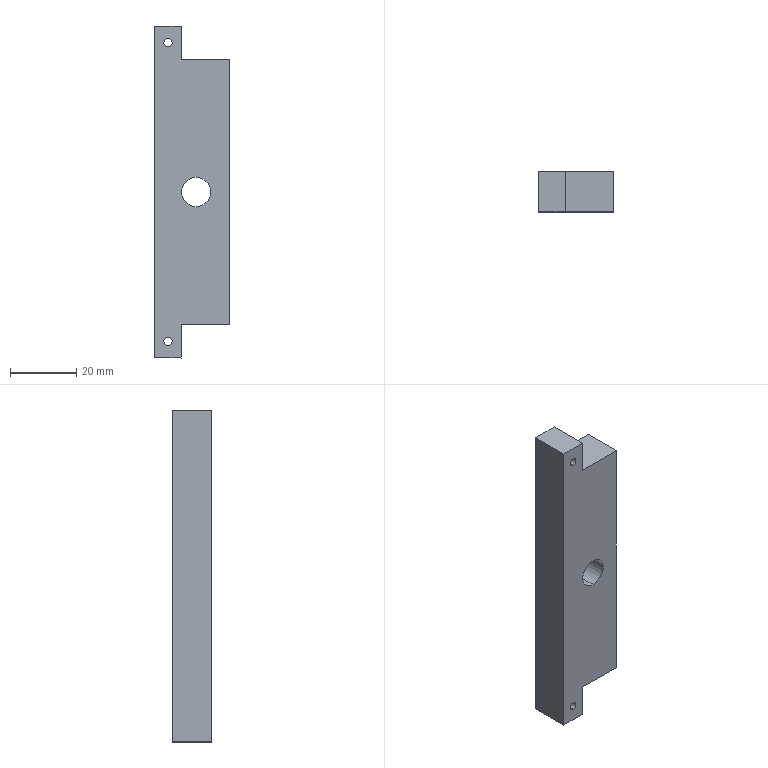Component | SolidWorks | LocatingDie-2_LocatingDieAdjustmentBlock-1 | 1 solid | 16 faces | box 22.5 x 12 x 100 mm | volume 22672 mm3 | plane 10 | cylinder 6 | commonest cylinder face diameters 2.5 x4 8.8 x2
build123d program:
from build123d import *

# Parameters (mm, degrees)
EXTRUDE1_DEPTH              = 12
M10X1_25_TAPPED_HOLE1_D     = 8.8
M10X1_25_TAPPED_HOLE1_DEPTH = 26.25
M10X1_25_TAPPED_HOLE1_TIP   = 2.644
M3_TAPPED_HOLE1_D           = 2.5
M3_TAPPED_HOLE1_DEPTH       = 25
M3_TAPPED_HOLE1_TIP         = 0.7511


with BuildPart() as part:
    # Sketch1 → Extrude1 (new body)
    with BuildSketch(Plane.XY):
        Polygon((-50, 4), (50, 4), (50, -4), (40, -4), (40, -18.5), (-40, -18.5), (-40, -4), (-50, -4), align=None)
    extrude(amount=EXTRUDE1_DEPTH)

    # M10x1.25 Tapped Hole1
    with Locations(Plane.XY.offset(12)):
        with Locations((0, -8.5)):
            Hole(M10X1_25_TAPPED_HOLE1_D / 2, depth=M10X1_25_TAPPED_HOLE1_DEPTH)
            with Locations((0, 0, -(M10X1_25_TAPPED_HOLE1_DEPTH + M10X1_25_TAPPED_HOLE1_TIP / 2))):  # 118° drill point
                Cone(0, M10X1_25_TAPPED_HOLE1_D / 2, M10X1_25_TAPPED_HOLE1_TIP, mode=Mode.SUBTRACT)

    # M3 Tapped Hole1
    with Locations(Plane.XY.offset(12)):
        with Locations((45, 0), (-45, 0)):
            Hole(M3_TAPPED_HOLE1_D / 2, depth=M3_TAPPED_HOLE1_DEPTH)
            with Locations((0, 0, -(M3_TAPPED_HOLE1_DEPTH + M3_TAPPED_HOLE1_TIP / 2))):  # 118° drill point
                Cone(0, M3_TAPPED_HOLE1_D / 2, M3_TAPPED_HOLE1_TIP, mode=Mode.SUBTRACT)


solid = part.part

# Placed as in the assembly
solid = solid.moved(Location((-305.284, 625.983, 14), (90, 0, 90)))
STEP:
#1=CARTESIAN_POINT('',(-12.019,24.645,2.274));
#2=VERTEX_POINT('',#1);
#3=CARTESIAN_POINT('',(-12.019,24.645,2.372));
#4=VERTEX_POINT('',#3);
#5=CARTESIAN_POINT('',(-12.019,24.645,2.323));
#6=DIRECTION('',(0.,-1.,0.));
#7=DIRECTION('',(0.,0.,1.));
#8=AXIS2_PLACEMENT_3D('',#5,#6,#7);
#9=CIRCLE('',#8,0.04921);
#10=EDGE_CURVE('',#2,#4,#9,.T.);
#11=ORIENTED_EDGE('',*,*,#10,.F.);
#12=CARTESIAN_POINT('',(-12.019,24.173,2.274));
#13=VERTEX_POINT('',#12);
#14=CARTESIAN_POINT('',(-12.019,24.173,2.274));
#15=DIRECTION('',(0.,-1.,0.));
#16=VECTOR('',#15,39.37);
#17=LINE('',#14,#16);
#18=EDGE_CURVE('',#2,#13,#17,.T.);
#19=ORIENTED_EDGE('',*,*,#18,.T.);
#20=CARTESIAN_POINT('',(-12.019,24.173,2.372));
#21=VERTEX_POINT('',#20);
#22=CARTESIAN_POINT('',(-12.019,24.173,2.323));
#23=DIRECTION('',(0.,-1.,0.));
#24=DIRECTION('',(0.,0.,1.));
#25=AXIS2_PLACEMENT_3D('',#22,#23,#24);
#26=CIRCLE('',#25,0.04921);
#27=EDGE_CURVE('',#13,#21,#26,.T.);
#28=ORIENTED_EDGE('',*,*,#27,.T.);
#29=CARTESIAN_POINT('',(-12.019,24.173,2.372));
#30=DIRECTION('',(0.,-1.,0.));
#31=VECTOR('',#30,39.37);
#32=LINE('',#29,#31);
#33=EDGE_CURVE('',#4,#21,#32,.T.);
#34=ORIENTED_EDGE('',*,*,#33,.F.);
#35=EDGE_LOOP('',(#11,#19,#28,#34));
#36=FACE_OUTER_BOUND('',#35,.T.);
#37=CARTESIAN_POINT('',(-12.019,24.173,2.323));
#38=DIRECTION('',(0.,-1.,0.));
#39=DIRECTION('',(0.,0.,1.));
#40=AXIS2_PLACEMENT_3D('',#37,#38,#39);
#41=CYLINDRICAL_SURFACE('',#40,0.04921);
#42=ADVANCED_FACE('',(#36),#41,.F.);
#43=CARTESIAN_POINT('',(-12.019,24.645,-1.27));
#44=VERTEX_POINT('',#43);
#45=CARTESIAN_POINT('',(-12.019,24.645,-1.171));
#46=VERTEX_POINT('',#45);
#47=CARTESIAN_POINT('',(-12.019,24.645,-1.22));
#48=DIRECTION('',(0.,-1.,0.));
#49=DIRECTION('',(0.,0.,1.));
#50=AXIS2_PLACEMENT_3D('',#47,#48,#49);
#51=CIRCLE('',#50,0.04921);
#52=EDGE_CURVE('',#44,#46,#51,.T.);
#53=ORIENTED_EDGE('',*,*,#52,.F.);
#54=CARTESIAN_POINT('',(-12.019,24.173,-1.27));
#55=VERTEX_POINT('',#54);
#56=CARTESIAN_POINT('',(-12.019,24.173,-1.27));
#57=DIRECTION('',(0.,-1.,0.));
#58=VECTOR('',#57,39.37);
#59=LINE('',#56,#58);
#60=EDGE_CURVE('',#44,#55,#59,.T.);
#61=ORIENTED_EDGE('',*,*,#60,.T.);
#62=CARTESIAN_POINT('',(-12.019,24.173,-1.171));
#63=VERTEX_POINT('',#62);
#64=CARTESIAN_POINT('',(-12.019,24.173,-1.22));
#65=DIRECTION('',(0.,-1.,0.));
#66=DIRECTION('',(0.,0.,1.));
#67=AXIS2_PLACEMENT_3D('',#64,#65,#66);
#68=CIRCLE('',#67,0.04921);
#69=EDGE_CURVE('',#55,#63,#68,.T.);
#70=ORIENTED_EDGE('',*,*,#69,.T.);
#71=CARTESIAN_POINT('',(-12.019,24.173,-1.171));
#72=DIRECTION('',(0.,-1.,0.));
#73=VECTOR('',#72,39.37);
#74=LINE('',#71,#73);
#75=EDGE_CURVE('',#46,#63,#74,.T.);
#76=ORIENTED_EDGE('',*,*,#75,.F.);
#77=EDGE_LOOP('',(#53,#61,#70,#76));
#78=FACE_OUTER_BOUND('',#77,.T.);
#79=CARTESIAN_POINT('',(-12.019,24.173,-1.22));
#80=DIRECTION('',(0.,-1.,0.));
#81=DIRECTION('',(0.,0.,1.));
#82=AXIS2_PLACEMENT_3D('',#79,#80,#81);
#83=CYLINDRICAL_SURFACE('',#82,0.04921);
#84=ADVANCED_FACE('',(#78),#83,.F.);
#85=CARTESIAN_POINT('',(-11.684,24.645,0.378));
#86=VERTEX_POINT('',#85);
#87=CARTESIAN_POINT('',(-11.684,24.645,0.7244));
#88=VERTEX_POINT('',#87);
#89=CARTESIAN_POINT('',(-11.684,24.645,0.5512));
#90=DIRECTION('',(0.,-1.,0.));
#91=DIRECTION('',(0.,0.,1.));
#92=AXIS2_PLACEMENT_3D('',#89,#90,#91);
#93=CIRCLE('',#92,0.1732);
#94=EDGE_CURVE('',#86,#88,#93,.T.);
#95=ORIENTED_EDGE('',*,*,#94,.F.);
#96=CARTESIAN_POINT('',(-11.684,24.173,0.378));
#97=VERTEX_POINT('',#96);
#98=CARTESIAN_POINT('',(-11.684,24.173,0.378));
#99=DIRECTION('',(0.,-1.,0.));
#100=VECTOR('',#99,39.37);
#101=LINE('',#98,#100);
#102=EDGE_CURVE('',#86,#97,#101,.T.);
#103=ORIENTED_EDGE('',*,*,#102,.T.);
#104=CARTESIAN_POINT('',(-11.684,24.173,0.7244));
#105=VERTEX_POINT('',#104);
#106=CARTESIAN_POINT('',(-11.684,24.173,0.5512));
#107=DIRECTION('',(0.,-1.,0.));
#108=DIRECTION('',(0.,0.,1.));
#109=AXIS2_PLACEMENT_3D('',#106,#107,#108);
#110=CIRCLE('',#109,0.1732);
#111=EDGE_CURVE('',#97,#105,#110,.T.);
#112=ORIENTED_EDGE('',*,*,#111,.T.);
#113=CARTESIAN_POINT('',(-11.684,24.173,0.7244));
#114=DIRECTION('',(0.,-1.,0.));
#115=VECTOR('',#114,39.37);
#116=LINE('',#113,#115);
#117=EDGE_CURVE('',#88,#105,#116,.T.);
#118=ORIENTED_EDGE('',*,*,#117,.F.);
#119=EDGE_LOOP('',(#95,#103,#112,#118));
#120=FACE_OUTER_BOUND('',#119,.T.);
#121=CARTESIAN_POINT('',(-11.684,24.173,0.5512));
#122=DIRECTION('',(0.,-1.,0.));
#123=DIRECTION('',(0.,0.,1.));
#124=AXIS2_PLACEMENT_3D('',#121,#122,#123);
#125=CYLINDRICAL_SURFACE('',#124,0.1732);
#126=ADVANCED_FACE('',(#120),#125,.F.);
#127=CARTESIAN_POINT('',(-12.177,24.645,-1.417));
#128=VERTEX_POINT('',#127);
#129=CARTESIAN_POINT('',(-11.862,24.645,-1.417));
#130=VERTEX_POINT('',#129);
#131=CARTESIAN_POINT('',(-12.177,24.645,-1.417));
#132=DIRECTION('',(1.,0.,-0.));
#133=VECTOR('',#132,39.37);
#134=LINE('',#131,#133);
#135=EDGE_CURVE('',#128,#130,#134,.T.);
#136=ORIENTED_EDGE('',*,*,#135,.T.);
#137=CARTESIAN_POINT('',(-11.862,24.173,-1.417));
#138=VERTEX_POINT('',#137);
#139=CARTESIAN_POINT('',(-11.862,24.173,-1.417));
#140=DIRECTION('',(-0.,1.,-0.));
#141=VECTOR('',#140,39.37);
#142=LINE('',#139,#141);
#143=EDGE_CURVE('',#138,#130,#142,.T.);
#144=ORIENTED_EDGE('',*,*,#143,.F.);
#145=CARTESIAN_POINT('',(-12.177,24.173,-1.417));
#146=VERTEX_POINT('',#145);
#147=CARTESIAN_POINT('',(-12.177,24.173,-1.417));
#148=DIRECTION('',(1.,0.,-0.));
#149=VECTOR('',#148,39.37);
#150=LINE('',#147,#149);
#151=EDGE_CURVE('',#146,#138,#150,.T.);
#152=ORIENTED_EDGE('',*,*,#151,.F.);
#153=CARTESIAN_POINT('',(-12.177,24.173,-1.417));
#154=DIRECTION('',(-0.,1.,-0.));
#155=VECTOR('',#154,39.37);
#156=LINE('',#153,#155);
#157=EDGE_CURVE('',#146,#128,#156,.T.);
#158=ORIENTED_EDGE('',*,*,#157,.T.);
#159=EDGE_LOOP('',(#136,#144,#152,#158));
#160=FACE_OUTER_BOUND('',#159,.T.);
#161=CARTESIAN_POINT('',(-12.177,24.173,-1.417));
#162=DIRECTION('',(0.,0.,1.));
#163=DIRECTION('',(-0.,1.,-0.));
#164=AXIS2_PLACEMENT_3D('',#161,#162,#163);
#165=PLANE('',#164);
#166=ADVANCED_FACE('',(#160),#165,.F.);
#167=CARTESIAN_POINT('',(-11.862,24.645,-1.024));
#168=VERTEX_POINT('',#167);
#169=CARTESIAN_POINT('',(-11.862,24.645,-1.417));
#170=DIRECTION('',(0.,0.,1.));
#171=VECTOR('',#170,39.37);
#172=LINE('',#169,#171);
#173=EDGE_CURVE('',#130,#168,#172,.T.);
#174=ORIENTED_EDGE('',*,*,#173,.T.);
#175=CARTESIAN_POINT('',(-11.862,24.173,-1.024));
#176=VERTEX_POINT('',#175);
#177=CARTESIAN_POINT('',(-11.862,24.173,-1.024));
#178=DIRECTION('',(-0.,1.,-0.));
#179=VECTOR('',#178,39.37);
#180=LINE('',#177,#179);
#181=EDGE_CURVE('',#176,#168,#180,.T.);
#182=ORIENTED_EDGE('',*,*,#181,.F.);
#183=CARTESIAN_POINT('',(-11.862,24.173,-1.417));
#184=DIRECTION('',(0.,0.,1.));
#185=VECTOR('',#184,39.37);
#186=LINE('',#183,#185);
#187=EDGE_CURVE('',#138,#176,#186,.T.);
#188=ORIENTED_EDGE('',*,*,#187,.F.);
#189=ORIENTED_EDGE('',*,*,#143,.T.);
#190=EDGE_LOOP('',(#174,#182,#188,#189));
#191=FACE_OUTER_BOUND('',#190,.T.);
#192=CARTESIAN_POINT('',(-11.862,24.173,-1.417));
#193=DIRECTION('',(-1.,-0.,0.));
#194=DIRECTION('',(0.,-1.,0.));
#195=AXIS2_PLACEMENT_3D('',#192,#193,#194);
#196=PLANE('',#195);
#197=ADVANCED_FACE('',(#191),#196,.F.);
#198=CARTESIAN_POINT('',(-11.291,24.645,-1.024));
#199=VERTEX_POINT('',#198);
#200=CARTESIAN_POINT('',(-11.862,24.645,-1.024));
#201=DIRECTION('',(1.,0.,-0.));
#202=VECTOR('',#201,39.37);
#203=LINE('',#200,#202);
#204=EDGE_CURVE('',#168,#199,#203,.T.);
#205=ORIENTED_EDGE('',*,*,#204,.T.);
#206=CARTESIAN_POINT('',(-11.291,24.173,-1.024));
#207=VERTEX_POINT('',#206);
#208=CARTESIAN_POINT('',(-11.291,24.173,-1.024));
#209=DIRECTION('',(-0.,1.,-0.));
#210=VECTOR('',#209,39.37);
#211=LINE('',#208,#210);
#212=EDGE_CURVE('',#207,#199,#211,.T.);
#213=ORIENTED_EDGE('',*,*,#212,.F.);
#214=CARTESIAN_POINT('',(-11.862,24.173,-1.024));
#215=DIRECTION('',(1.,0.,-0.));
#216=VECTOR('',#215,39.37);
#217=LINE('',#214,#216);
#218=EDGE_CURVE('',#176,#207,#217,.T.);
#219=ORIENTED_EDGE('',*,*,#218,.F.);
#220=ORIENTED_EDGE('',*,*,#181,.T.);
#221=EDGE_LOOP('',(#205,#213,#219,#220));
#222=FACE_OUTER_BOUND('',#221,.T.);
#223=CARTESIAN_POINT('',(-11.862,24.173,-1.024));
#224=DIRECTION('',(0.,0.,1.));
#225=DIRECTION('',(-1.,-0.,0.));
#226=AXIS2_PLACEMENT_3D('',#223,#224,#225);
#227=PLANE('',#226);
#228=ADVANCED_FACE('',(#222),#227,.F.);
#229=CARTESIAN_POINT('',(-11.291,24.645,2.126));
#230=VERTEX_POINT('',#229);
#231=CARTESIAN_POINT('',(-11.291,24.645,-1.024));
#232=DIRECTION('',(0.,0.,1.));
#233=VECTOR('',#232,39.37);
#234=LINE('',#231,#233);
#235=EDGE_CURVE('',#199,#230,#234,.T.);
#236=ORIENTED_EDGE('',*,*,#235,.T.);
#237=CARTESIAN_POINT('',(-11.291,24.173,2.126));
#238=VERTEX_POINT('',#237);
#239=CARTESIAN_POINT('',(-11.291,24.173,2.126));
#240=DIRECTION('',(-0.,1.,-0.));
#241=VECTOR('',#240,39.37);
#242=LINE('',#239,#241);
#243=EDGE_CURVE('',#238,#230,#242,.T.);
#244=ORIENTED_EDGE('',*,*,#243,.F.);
#245=CARTESIAN_POINT('',(-11.291,24.173,-1.024));
#246=DIRECTION('',(0.,0.,1.));
#247=VECTOR('',#246,39.37);
#248=LINE('',#245,#247);
#249=EDGE_CURVE('',#207,#238,#248,.T.);
#250=ORIENTED_EDGE('',*,*,#249,.F.);
#251=ORIENTED_EDGE('',*,*,#212,.T.);
#252=EDGE_LOOP('',(#236,#244,#250,#251));
#253=FACE_OUTER_BOUND('',#252,.T.);
#254=CARTESIAN_POINT('',(-11.291,24.173,-1.024));
#255=DIRECTION('',(-1.,-0.,0.));
#256=DIRECTION('',(0.,-1.,0.));
#257=AXIS2_PLACEMENT_3D('',#254,#255,#256);
#258=PLANE('',#257);
#259=ADVANCED_FACE('',(#253),#258,.F.);
#260=CARTESIAN_POINT('',(-11.862,24.645,2.126));
#261=VERTEX_POINT('',#260);
#262=CARTESIAN_POINT('',(-11.862,24.645,2.126));
#263=DIRECTION('',(-1.,-0.,0.));
#264=VECTOR('',#263,39.37);
#265=LINE('',#262,#264);
#266=EDGE_CURVE('',#230,#261,#265,.T.);
#267=ORIENTED_EDGE('',*,*,#266,.T.);
#268=CARTESIAN_POINT('',(-11.862,24.173,2.126));
#269=VERTEX_POINT('',#268);
#270=CARTESIAN_POINT('',(-11.862,24.173,2.126));
#271=DIRECTION('',(-0.,1.,-0.));
#272=VECTOR('',#271,39.37);
#273=LINE('',#270,#272);
#274=EDGE_CURVE('',#269,#261,#273,.T.);
#275=ORIENTED_EDGE('',*,*,#274,.F.);
#276=CARTESIAN_POINT('',(-11.862,24.173,2.126));
#277=DIRECTION('',(-1.,-0.,0.));
#278=VECTOR('',#277,39.37);
#279=LINE('',#276,#278);
#280=EDGE_CURVE('',#238,#269,#279,.T.);
#281=ORIENTED_EDGE('',*,*,#280,.F.);
#282=ORIENTED_EDGE('',*,*,#243,.T.);
#283=EDGE_LOOP('',(#267,#275,#281,#282));
#284=FACE_OUTER_BOUND('',#283,.T.);
#285=CARTESIAN_POINT('',(-11.862,24.173,2.126));
#286=DIRECTION('',(-0.,-0.,-1.));
#287=DIRECTION('',(0.,-1.,0.));
#288=AXIS2_PLACEMENT_3D('',#285,#286,#287);
#289=PLANE('',#288);
#290=ADVANCED_FACE('',(#284),#289,.F.);
#291=CARTESIAN_POINT('',(-11.862,24.645,2.52));
#292=VERTEX_POINT('',#291);
#293=CARTESIAN_POINT('',(-11.862,24.645,2.126));
#294=DIRECTION('',(0.,0.,1.));
#295=VECTOR('',#294,39.37);
#296=LINE('',#293,#295);
#297=EDGE_CURVE('',#261,#292,#296,.T.);
#298=ORIENTED_EDGE('',*,*,#297,.T.);
#299=CARTESIAN_POINT('',(-11.862,24.173,2.52));
#300=VERTEX_POINT('',#299);
#301=CARTESIAN_POINT('',(-11.862,24.173,2.52));
#302=DIRECTION('',(-0.,1.,-0.));
#303=VECTOR('',#302,39.37);
#304=LINE('',#301,#303);
#305=EDGE_CURVE('',#300,#292,#304,.T.);
#306=ORIENTED_EDGE('',*,*,#305,.F.);
#307=CARTESIAN_POINT('',(-11.862,24.173,2.126));
#308=DIRECTION('',(0.,0.,1.));
#309=VECTOR('',#308,39.37);
#310=LINE('',#307,#309);
#311=EDGE_CURVE('',#269,#300,#310,.T.);
#312=ORIENTED_EDGE('',*,*,#311,.F.);
#313=ORIENTED_EDGE('',*,*,#274,.T.);
#314=EDGE_LOOP('',(#298,#306,#312,#313));
#315=FACE_OUTER_BOUND('',#314,.T.);
#316=CARTESIAN_POINT('',(-11.862,24.173,2.126));
#317=DIRECTION('',(-1.,-0.,0.));
#318=DIRECTION('',(0.,-1.,0.));
#319=AXIS2_PLACEMENT_3D('',#316,#317,#318);
#320=PLANE('',#319);
#321=ADVANCED_FACE('',(#315),#320,.F.);
#322=CARTESIAN_POINT('',(-12.177,24.645,2.52));
#323=VERTEX_POINT('',#322);
#324=CARTESIAN_POINT('',(-12.177,24.645,2.52));
#325=DIRECTION('',(-1.,-0.,0.));
#326=VECTOR('',#325,39.37);
#327=LINE('',#324,#326);
#328=EDGE_CURVE('',#292,#323,#327,.T.);
#329=ORIENTED_EDGE('',*,*,#328,.T.);
#330=CARTESIAN_POINT('',(-12.177,24.173,2.52));
#331=VERTEX_POINT('',#330);
#332=CARTESIAN_POINT('',(-12.177,24.173,2.52));
#333=DIRECTION('',(-0.,1.,-0.));
#334=VECTOR('',#333,39.37);
#335=LINE('',#332,#334);
#336=EDGE_CURVE('',#331,#323,#335,.T.);
#337=ORIENTED_EDGE('',*,*,#336,.F.);
#338=CARTESIAN_POINT('',(-12.177,24.173,2.52));
#339=DIRECTION('',(-1.,-0.,0.));
#340=VECTOR('',#339,39.37);
#341=LINE('',#338,#340);
#342=EDGE_CURVE('',#300,#331,#341,.T.);
#343=ORIENTED_EDGE('',*,*,#342,.F.);
#344=ORIENTED_EDGE('',*,*,#305,.T.);
#345=EDGE_LOOP('',(#329,#337,#343,#344));
#346=FACE_OUTER_BOUND('',#345,.T.);
#347=CARTESIAN_POINT('',(-12.177,24.173,2.52));
#348=DIRECTION('',(-0.,-0.,-1.));
#349=DIRECTION('',(0.,-1.,0.));
#350=AXIS2_PLACEMENT_3D('',#347,#348,#349);
#351=PLANE('',#350);
#352=ADVANCED_FACE('',(#346),#351,.F.);
#353=CARTESIAN_POINT('',(-12.177,24.645,-1.417));
#354=DIRECTION('',(-0.,-0.,-1.));
#355=VECTOR('',#354,39.37);
#356=LINE('',#353,#355);
#357=EDGE_CURVE('',#323,#128,#356,.T.);
#358=ORIENTED_EDGE('',*,*,#357,.T.);
#359=ORIENTED_EDGE('',*,*,#157,.F.);
#360=CARTESIAN_POINT('',(-12.177,24.173,-1.417));
#361=DIRECTION('',(-0.,-0.,-1.));
#362=VECTOR('',#361,39.37);
#363=LINE('',#360,#362);
#364=EDGE_CURVE('',#331,#146,#363,.T.);
#365=ORIENTED_EDGE('',*,*,#364,.F.);
#366=ORIENTED_EDGE('',*,*,#336,.T.);
#367=EDGE_LOOP('',(#358,#359,#365,#366));
#368=FACE_OUTER_BOUND('',#367,.T.);
#369=CARTESIAN_POINT('',(-12.177,24.173,-1.417));
#370=DIRECTION('',(1.,0.,-0.));
#371=DIRECTION('',(-0.,1.,-0.));
#372=AXIS2_PLACEMENT_3D('',#369,#370,#371);
#373=PLANE('',#372);
#374=ADVANCED_FACE('',(#368),#373,.F.);
#375=CARTESIAN_POINT('',(-12.019,24.173,2.323));
#376=DIRECTION('',(0.,-1.,0.));
#377=DIRECTION('',(0.,0.,1.));
#378=AXIS2_PLACEMENT_3D('',#375,#376,#377);
#379=CIRCLE('',#378,0.04921);
#380=EDGE_CURVE('',#21,#13,#379,.T.);
#381=ORIENTED_EDGE('',*,*,#380,.F.);
#382=ORIENTED_EDGE('',*,*,#27,.F.);
#383=EDGE_LOOP('',(#381,#382));
#384=FACE_BOUND('',#383,.T.);
#385=CARTESIAN_POINT('',(-12.019,24.173,-1.22));
#386=DIRECTION('',(0.,-1.,0.));
#387=DIRECTION('',(0.,0.,1.));
#388=AXIS2_PLACEMENT_3D('',#385,#386,#387);
#389=CIRCLE('',#388,0.04921);
#390=EDGE_CURVE('',#63,#55,#389,.T.);
#391=ORIENTED_EDGE('',*,*,#390,.F.);
#392=ORIENTED_EDGE('',*,*,#69,.F.);
#393=EDGE_LOOP('',(#391,#392));
#394=FACE_BOUND('',#393,.T.);
#395=CARTESIAN_POINT('',(-11.684,24.173,0.5512));
#396=DIRECTION('',(0.,-1.,0.));
#397=DIRECTION('',(0.,0.,1.));
#398=AXIS2_PLACEMENT_3D('',#395,#396,#397);
#399=CIRCLE('',#398,0.1732);
#400=EDGE_CURVE('',#105,#97,#399,.T.);
#401=ORIENTED_EDGE('',*,*,#400,.F.);
#402=ORIENTED_EDGE('',*,*,#111,.F.);
#403=EDGE_LOOP('',(#401,#402));
#404=FACE_BOUND('',#403,.T.);
#405=ORIENTED_EDGE('',*,*,#151,.T.);
#406=ORIENTED_EDGE('',*,*,#187,.T.);
#407=ORIENTED_EDGE('',*,*,#218,.T.);
#408=ORIENTED_EDGE('',*,*,#249,.T.);
#409=ORIENTED_EDGE('',*,*,#280,.T.);
#410=ORIENTED_EDGE('',*,*,#311,.T.);
#411=ORIENTED_EDGE('',*,*,#342,.T.);
#412=ORIENTED_EDGE('',*,*,#364,.T.);
#413=EDGE_LOOP('',(#405,#406,#407,#408,#409,#410,#411,#412));
#414=FACE_OUTER_BOUND('',#413,.T.);
#415=CARTESIAN_POINT('',(-11.862,24.173,-1.417));
#416=DIRECTION('',(0.,-1.,0.));
#417=DIRECTION('',(0.,0.,1.));
#418=AXIS2_PLACEMENT_3D('',#415,#416,#417);
#419=PLANE('',#418);
#420=ADVANCED_FACE('',(#384,#394,#404,#414),#419,.T.);
#421=CARTESIAN_POINT('',(-12.019,24.645,2.323));
#422=DIRECTION('',(0.,-1.,0.));
#423=DIRECTION('',(0.,0.,1.));
#424=AXIS2_PLACEMENT_3D('',#421,#422,#423);
#425=CIRCLE('',#424,0.04921);
#426=EDGE_CURVE('',#4,#2,#425,.T.);
#427=ORIENTED_EDGE('',*,*,#426,.T.);
#428=ORIENTED_EDGE('',*,*,#10,.T.);
#429=EDGE_LOOP('',(#427,#428));
#430=FACE_BOUND('',#429,.T.);
#431=CARTESIAN_POINT('',(-12.019,24.645,-1.22));
#432=DIRECTION('',(0.,-1.,0.));
#433=DIRECTION('',(0.,0.,1.));
#434=AXIS2_PLACEMENT_3D('',#431,#432,#433);
#435=CIRCLE('',#434,0.04921);
#436=EDGE_CURVE('',#46,#44,#435,.T.);
#437=ORIENTED_EDGE('',*,*,#436,.T.);
#438=ORIENTED_EDGE('',*,*,#52,.T.);
#439=EDGE_LOOP('',(#437,#438));
#440=FACE_BOUND('',#439,.T.);
#441=CARTESIAN_POINT('',(-11.684,24.645,0.5512));
#442=DIRECTION('',(0.,-1.,0.));
#443=DIRECTION('',(0.,0.,1.));
#444=AXIS2_PLACEMENT_3D('',#441,#442,#443);
#445=CIRCLE('',#444,0.1732);
#446=EDGE_CURVE('',#88,#86,#445,.T.);
#447=ORIENTED_EDGE('',*,*,#446,.T.);
#448=ORIENTED_EDGE('',*,*,#94,.T.);
#449=EDGE_LOOP('',(#447,#448));
#450=FACE_BOUND('',#449,.T.);
#451=ORIENTED_EDGE('',*,*,#135,.F.);
#452=ORIENTED_EDGE('',*,*,#357,.F.);
#453=ORIENTED_EDGE('',*,*,#328,.F.);
#454=ORIENTED_EDGE('',*,*,#297,.F.);
#455=ORIENTED_EDGE('',*,*,#266,.F.);
#456=ORIENTED_EDGE('',*,*,#235,.F.);
#457=ORIENTED_EDGE('',*,*,#204,.F.);
#458=ORIENTED_EDGE('',*,*,#173,.F.);
#459=EDGE_LOOP('',(#451,#452,#453,#454,#455,#456,#457,#458));
#460=FACE_OUTER_BOUND('',#459,.T.);
#461=CARTESIAN_POINT('',(-11.862,24.645,-1.417));
#462=DIRECTION('',(0.,-1.,0.));
#463=DIRECTION('',(0.,0.,1.));
#464=AXIS2_PLACEMENT_3D('',#461,#462,#463);
#465=PLANE('',#464);
#466=ADVANCED_FACE('',(#430,#440,#450,#460),#465,.F.);
#467=ORIENTED_EDGE('',*,*,#102,.F.);
#468=ORIENTED_EDGE('',*,*,#446,.F.);
#469=ORIENTED_EDGE('',*,*,#117,.T.);
#470=ORIENTED_EDGE('',*,*,#400,.T.);
#471=EDGE_LOOP('',(#467,#468,#469,#470));
#472=FACE_OUTER_BOUND('',#471,.T.);
#473=CARTESIAN_POINT('',(-11.684,24.173,0.5512));
#474=DIRECTION('',(0.,-1.,0.));
#475=DIRECTION('',(0.,0.,1.));
#476=AXIS2_PLACEMENT_3D('',#473,#474,#475);
#477=CYLINDRICAL_SURFACE('',#476,0.1732);
#478=ADVANCED_FACE('',(#472),#477,.F.);
#479=ORIENTED_EDGE('',*,*,#60,.F.);
#480=ORIENTED_EDGE('',*,*,#436,.F.);
#481=ORIENTED_EDGE('',*,*,#75,.T.);
#482=ORIENTED_EDGE('',*,*,#390,.T.);
#483=EDGE_LOOP('',(#479,#480,#481,#482));
#484=FACE_OUTER_BOUND('',#483,.T.);
#485=CARTESIAN_POINT('',(-12.019,24.173,-1.22));
#486=DIRECTION('',(0.,-1.,0.));
#487=DIRECTION('',(0.,0.,1.));
#488=AXIS2_PLACEMENT_3D('',#485,#486,#487);
#489=CYLINDRICAL_SURFACE('',#488,0.04921);
#490=ADVANCED_FACE('',(#484),#489,.F.);
#491=ORIENTED_EDGE('',*,*,#18,.F.);
#492=ORIENTED_EDGE('',*,*,#426,.F.);
#493=ORIENTED_EDGE('',*,*,#33,.T.);
#494=ORIENTED_EDGE('',*,*,#380,.T.);
#495=EDGE_LOOP('',(#491,#492,#493,#494));
#496=FACE_OUTER_BOUND('',#495,.T.);
#497=CARTESIAN_POINT('',(-12.019,24.173,2.323));
#498=DIRECTION('',(0.,-1.,0.));
#499=DIRECTION('',(0.,0.,1.));
#500=AXIS2_PLACEMENT_3D('',#497,#498,#499);
#501=CYLINDRICAL_SURFACE('',#500,0.04921);
#502=ADVANCED_FACE('',(#496),#501,.F.);
#503=CLOSED_SHELL('',(#42,#84,#126,#166,#197,#228,#259,#290,#321,#352,#374,#420,#466,#478,#490,#502));
#504=MANIFOLD_SOLID_BREP('',#503);
#505=CARTESIAN_POINT('',(0.,0.,0.));
#506=DIRECTION('',(0.,0.,1.));
#507=DIRECTION('',(1.,0.,0.));
#508=AXIS2_PLACEMENT_3D('',#505,#506,#507);
#509=(LENGTH_UNIT()NAMED_UNIT(*)SI_UNIT($,.METRE.));
#510=LENGTH_MEASURE_WITH_UNIT(LENGTH_MEASURE(0.0254),#509);
#511=DIMENSIONAL_EXPONENTS(1.,0.,0.,0.,0.,0.,0.);
#512=(CONVERSION_BASED_UNIT('',#510)LENGTH_UNIT()NAMED_UNIT(#511));
#513=UNCERTAINTY_MEASURE_WITH_UNIT(LENGTH_MEASURE(0.00001),#512,'','');
#514=(NAMED_UNIT(*)PLANE_ANGLE_UNIT()SI_UNIT($,.RADIAN.));
#515=(NAMED_UNIT(*)SI_UNIT($,.STERADIAN.)SOLID_ANGLE_UNIT());
#516=(GEOMETRIC_REPRESENTATION_CONTEXT(3)GLOBAL_UNCERTAINTY_ASSIGNED_CONTEXT((#513))GLOBAL_UNIT_ASSIGNED_CONTEXT((#512,#514,#515))REPRESENTATION_CONTEXT('',''));
#517=ADVANCED_BREP_SHAPE_REPRESENTATION('',(#504,#508),#516);
#518=COLOUR_RGB('',0.7922,0.8196,0.9333);
#519=FILL_AREA_STYLE_COLOUR('',#518);
#520=FILL_AREA_STYLE('',(#519));
#521=SURFACE_STYLE_FILL_AREA(#520);
#522=SURFACE_SIDE_STYLE('',(#521));
#523=SURFACE_STYLE_USAGE(.BOTH.,#522);
#524=PRESENTATION_STYLE_ASSIGNMENT((#523));
#525=STYLED_ITEM('',(#524),#504);
#526=(LENGTH_UNIT()NAMED_UNIT(*)SI_UNIT($,.METRE.));
#527=LENGTH_MEASURE_WITH_UNIT(LENGTH_MEASURE(0.0254),#526);
#528=DIMENSIONAL_EXPONENTS(1.,0.,0.,0.,0.,0.,0.);
#529=(CONVERSION_BASED_UNIT('',#527)LENGTH_UNIT()NAMED_UNIT(#528));
#530=UNCERTAINTY_MEASURE_WITH_UNIT(LENGTH_MEASURE(0.00001),#529,'','');
#531=(NAMED_UNIT(*)PLANE_ANGLE_UNIT()SI_UNIT($,.RADIAN.));
#532=(NAMED_UNIT(*)SI_UNIT($,.STERADIAN.)SOLID_ANGLE_UNIT());
#533=(GEOMETRIC_REPRESENTATION_CONTEXT(3)GLOBAL_UNCERTAINTY_ASSIGNED_CONTEXT((#530))GLOBAL_UNIT_ASSIGNED_CONTEXT((#529,#531,#532))REPRESENTATION_CONTEXT('',''));
#534=MECHANICAL_DESIGN_GEOMETRIC_PRESENTATION_REPRESENTATION('',(#525),#533);
#535=PRESENTATION_LAYER_ASSIGNMENT('','',(#525));